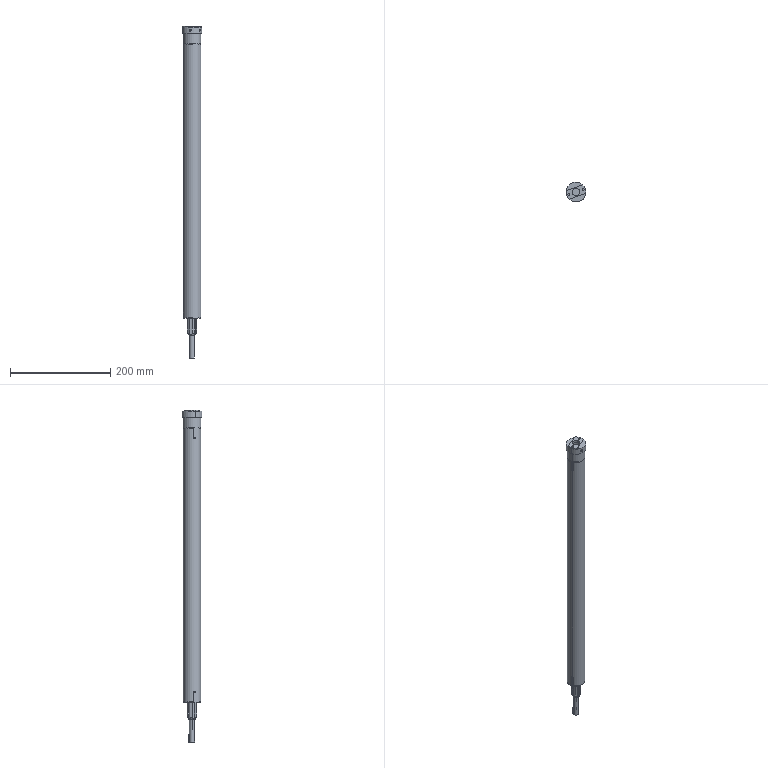Component | SolidWorks | Motor-2 | 4 solids | 117 faces | volume 566554 mm3 | plane 64 | cylinder 46 | cone 7 | commonest cylinder face diameters 4 x12 14 x7 35 x6 20 x4 2 x4 39 x3 14.5 x2 35.4 x2